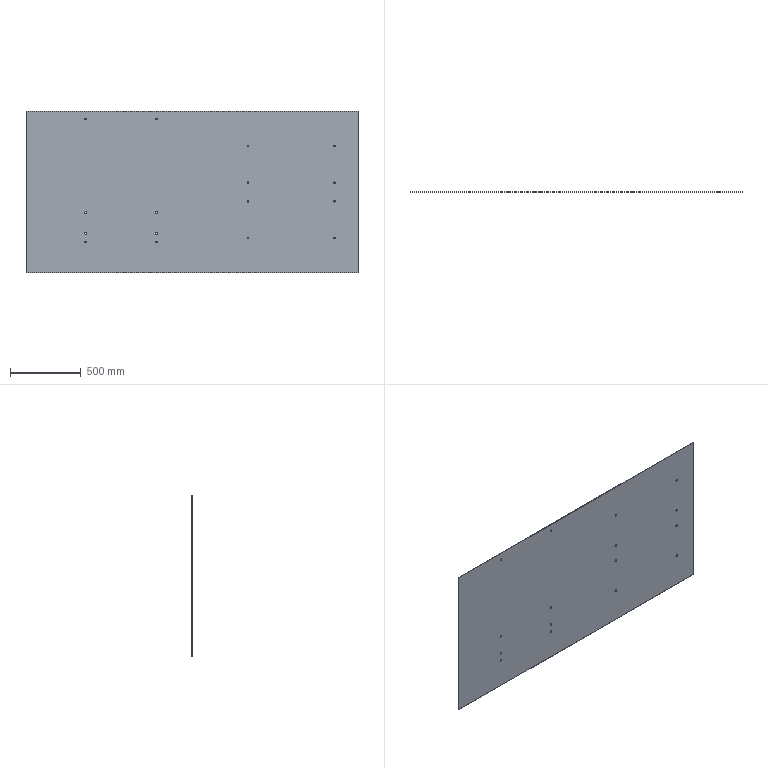Component | SolidWorks | 43BottomPlate-1 | 1 solid | 38 faces | box 2340 x 3 x 1140 mm | volume 7997371 mm3 | cylinder 32 | plane 6 | commonest cylinder face diameters 12 x32
build123d program:
from build123d import *

# Parameters (mm, degrees)
SKETCH1_W                  = 2340
SKETCH1_H                  = 1140
BOSS_EXTRUDE1_DEPTH        = 3
F_12_0_12_DIAMETER_HOLE1_D = 12


with BuildPart() as part:
    # Sketch1 → Boss-Extrude1 (new body)
    with BuildSketch(Plane(origin=(0, 0, 0), x_dir=(1, 0, 0), z_dir=(0, 1, 0))):
        with Locations((1101.698, 550.965)):
            Rectangle(SKETCH1_W, SKETCH1_H)
    extrude(amount=BOSS_EXTRUDE1_DEPTH)

    # 12.0 _12_ Diameter Hole1 (through all)
    with Locations(Plane(origin=(0, 3, 0), x_dir=(-1, 0, 0), z_dir=(0, 1, 0))):
        with Locations((-351.698, -902.965), (-351.698, -842.965), (-351.698, -695.965), (-351.698, -35.965), (-2104.198, -225.965), (-2104.198, -485.965), (-2104.198, -615.965), (-2104.198, -875.965), (-1497.198, -225.965), (-1497.198, -485.965), (-1497.198, -615.965), (-1497.198, -875.965), (-851.698, -902.965), (-851.698, -842.965), (-851.698, -695.965), (-851.698, -35.965)):
            Hole(F_12_0_12_DIAMETER_HOLE1_D / 2)


solid = part.part

# Placed as in the assembly
solid = solid.moved(Location((-25.226, -39.54, 1188.073), (0, 0, 0)))